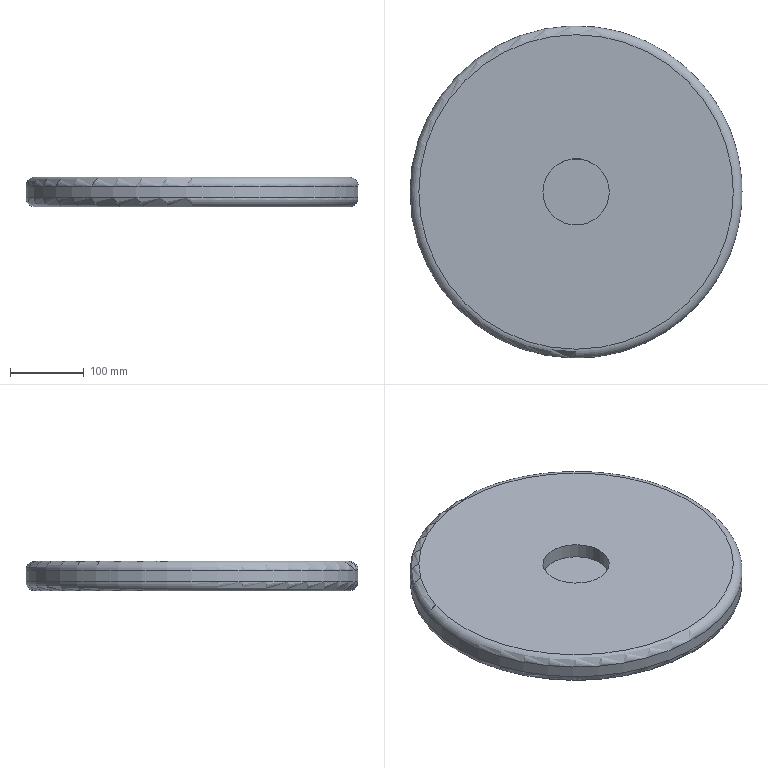Component | NX | BASE | 1 solid | 7 faces | box 450 x 450 x 40 mm | volume 6148156 mm3 | plane 3 | cylinder 2 | torus 2 | commonest cylinder face diameters 450 x1 90 x1
STEP:
#1=CARTESIAN_POINT('',(0.,0.,0.));
#2=DIRECTION('',(0.,0.,1.));
#3=DIRECTION('',(1.,0.,0.));
#4=AXIS2_PLACEMENT_3D('',#1,#2,#3);
#5=CARTESIAN_POINT('',(-225.,-0.,-1130.5));
#6=VERTEX_POINT('',#5);
#7=CARTESIAN_POINT('',(0.,-0.,-1130.5));
#8=DIRECTION('',(0.,0.,1.));
#9=DIRECTION('',(-1.,0.,0.));
#10=AXIS2_PLACEMENT_3D('',#7,#8,#9);
#11=CIRCLE('',#10,225.);
#12=CARTESIAN_POINT('',(0.,-0.,-1102.5));
#13=DIRECTION('',(0.,0.,-1.));
#14=DIRECTION('',(-1.,0.,0.));
#15=AXIS2_PLACEMENT_3D('',#12,#13,#14);
#16=CYLINDRICAL_SURFACE('',#15,225.);
#17=CARTESIAN_POINT('',(6.283,28.));
#18=DIRECTION('',(-1.,0.));
#19=VECTOR('',#18,1.);
#20=LINE('',#17,#19);
#21=(GEOMETRIC_REPRESENTATION_CONTEXT(2)PARAMETRIC_REPRESENTATION_CONTEXT()REPRESENTATION_CONTEXT('',''));
#22=DEFINITIONAL_REPRESENTATION('',(#20),#21);
#23=PCURVE('',#16,#22);
#24=CARTESIAN_POINT('',(0.,-0.,-1130.5));
#25=DIRECTION('',(0.,0.,-1.));
#26=DIRECTION('',(-1.,0.,0.));
#27=AXIS2_PLACEMENT_3D('',#24,#25,#26);
#28=TOROIDAL_SURFACE('',#27,213.,12.);
#29=CARTESIAN_POINT('',(6.283,6.283));
#30=DIRECTION('',(-1.,0.));
#31=VECTOR('',#30,1.);
#32=LINE('',#29,#31);
#33=(GEOMETRIC_REPRESENTATION_CONTEXT(2)PARAMETRIC_REPRESENTATION_CONTEXT()REPRESENTATION_CONTEXT('',''));
#34=DEFINITIONAL_REPRESENTATION('',(#32),#33);
#35=PCURVE('',#28,#34);
#36=SURFACE_CURVE('',#11,(#23,#35),.PCURVE_S1.);
#37=EDGE_CURVE('',#6,#6,#36,.T.);
#38=ORIENTED_EDGE('',*,*,#37,.T.);
#39=CARTESIAN_POINT('',(-225.,-0.,-1114.5));
#40=VERTEX_POINT('',#39);
#41=CARTESIAN_POINT('',(-225.,-0.,-1114.5));
#42=CARTESIAN_POINT('',(-225.,-0.,-1130.5));
#43=B_SPLINE_CURVE_WITH_KNOTS('',1,(#41,#42),.UNSPECIFIED.,.F.,.F.,(2,2),(12.,28.),.PIECEWISE_BEZIER_KNOTS.);
#44=CARTESIAN_POINT('',(0.,0.));
#45=DIRECTION('',(0.,1.));
#46=VECTOR('',#45,1.);
#47=LINE('',#44,#46);
#48=(GEOMETRIC_REPRESENTATION_CONTEXT(2)PARAMETRIC_REPRESENTATION_CONTEXT()REPRESENTATION_CONTEXT('',''));
#49=DEFINITIONAL_REPRESENTATION('',(#47),#48);
#50=PCURVE('',#16,#49);
#51=CARTESIAN_POINT('',(6.283,0.));
#52=DIRECTION('',(0.,1.));
#53=VECTOR('',#52,1.);
#54=LINE('',#51,#53);
#55=(GEOMETRIC_REPRESENTATION_CONTEXT(2)PARAMETRIC_REPRESENTATION_CONTEXT()REPRESENTATION_CONTEXT('',''));
#56=DEFINITIONAL_REPRESENTATION('',(#54),#55);
#57=PCURVE('',#16,#56);
#58=SEAM_CURVE('',#43,(#50,#57),.PCURVE_S1.);
#59=EDGE_CURVE('',#40,#6,#58,.T.);
#60=ORIENTED_EDGE('',*,*,#59,.F.);
#61=CARTESIAN_POINT('',(0.,-0.,-1114.5));
#62=DIRECTION('',(0.,0.,-1.));
#63=DIRECTION('',(-1.,0.,0.));
#64=AXIS2_PLACEMENT_3D('',#61,#62,#63);
#65=CIRCLE('',#64,225.);
#66=CARTESIAN_POINT('',(0.,12.));
#67=DIRECTION('',(1.,0.));
#68=VECTOR('',#67,1.);
#69=LINE('',#66,#68);
#70=(GEOMETRIC_REPRESENTATION_CONTEXT(2)PARAMETRIC_REPRESENTATION_CONTEXT()REPRESENTATION_CONTEXT('',''));
#71=DEFINITIONAL_REPRESENTATION('',(#69),#70);
#72=PCURVE('',#16,#71);
#73=CARTESIAN_POINT('',(0.,-0.,-1114.5));
#74=DIRECTION('',(0.,0.,-1.));
#75=DIRECTION('',(-1.,0.,0.));
#76=AXIS2_PLACEMENT_3D('',#73,#74,#75);
#77=TOROIDAL_SURFACE('',#76,213.,12.);
#78=CARTESIAN_POINT('',(0.,6.283));
#79=DIRECTION('',(1.,0.));
#80=VECTOR('',#79,1.);
#81=LINE('',#78,#80);
#82=(GEOMETRIC_REPRESENTATION_CONTEXT(2)PARAMETRIC_REPRESENTATION_CONTEXT()REPRESENTATION_CONTEXT('',''));
#83=DEFINITIONAL_REPRESENTATION('',(#81),#82);
#84=PCURVE('',#77,#83);
#85=SURFACE_CURVE('',#65,(#72,#84),.PCURVE_S1.);
#86=EDGE_CURVE('',#40,#40,#85,.T.);
#87=ORIENTED_EDGE('',*,*,#86,.T.);
#88=ORIENTED_EDGE('',*,*,#59,.T.);
#89=EDGE_LOOP('',(#38,#60,#87,#88));
#90=FACE_BOUND('',#89,.T.);
#91=ADVANCED_FACE('',(#90),#16,.T.);
#92=CARTESIAN_POINT('',(45.,-0.,-1102.5));
#93=VERTEX_POINT('',#92);
#94=CARTESIAN_POINT('',(0.,-0.,-1102.5));
#95=DIRECTION('',(0.,0.,-1.));
#96=DIRECTION('',(1.,0.,0.));
#97=AXIS2_PLACEMENT_3D('',#94,#95,#96);
#98=CIRCLE('',#97,45.);
#99=CARTESIAN_POINT('',(0.,-0.,-1102.5));
#100=DIRECTION('',(0.,0.,-1.));
#101=DIRECTION('',(-1.,0.,0.));
#102=AXIS2_PLACEMENT_3D('',#99,#100,#101);
#103=PLANE('',#102);
#104=CARTESIAN_POINT('',(0.,0.));
#105=DIRECTION('',(-1.,0.));
#106=AXIS2_PLACEMENT_2D('',#104,#105);
#107=CIRCLE('',#106,45.);
#108=(GEOMETRIC_REPRESENTATION_CONTEXT(2)PARAMETRIC_REPRESENTATION_CONTEXT()REPRESENTATION_CONTEXT('',''));
#109=DEFINITIONAL_REPRESENTATION('',(#107),#108);
#110=PCURVE('',#103,#109);
#111=CARTESIAN_POINT('',(0.,-0.,-1122.5));
#112=DIRECTION('',(0.,0.,1.));
#113=DIRECTION('',(1.,0.,0.));
#114=AXIS2_PLACEMENT_3D('',#111,#112,#113);
#115=CYLINDRICAL_SURFACE('',#114,45.);
#116=CARTESIAN_POINT('',(6.283,20.));
#117=DIRECTION('',(-1.,0.));
#118=VECTOR('',#117,1.);
#119=LINE('',#116,#118);
#120=(GEOMETRIC_REPRESENTATION_CONTEXT(2)PARAMETRIC_REPRESENTATION_CONTEXT()REPRESENTATION_CONTEXT('',''));
#121=DEFINITIONAL_REPRESENTATION('',(#119),#120);
#122=PCURVE('',#115,#121);
#123=SURFACE_CURVE('',#98,(#110,#122),.PCURVE_S1.);
#124=EDGE_CURVE('',#93,#93,#123,.T.);
#125=ORIENTED_EDGE('',*,*,#124,.T.);
#126=EDGE_LOOP('',(#125));
#127=FACE_BOUND('',#126,.T.);
#128=CARTESIAN_POINT('',(-213.,-0.,-1102.5));
#129=VERTEX_POINT('',#128);
#130=CARTESIAN_POINT('',(0.,-0.,-1102.5));
#131=DIRECTION('',(0.,0.,1.));
#132=DIRECTION('',(-1.,0.,0.));
#133=AXIS2_PLACEMENT_3D('',#130,#131,#132);
#134=CIRCLE('',#133,213.);
#135=CARTESIAN_POINT('',(213.,0.));
#136=CARTESIAN_POINT('',(213.,-368.927));
#137=CARTESIAN_POINT('',(-106.5,-184.463));
#138=CARTESIAN_POINT('',(-426.,-0.));
#139=CARTESIAN_POINT('',(-106.5,184.463));
#140=CARTESIAN_POINT('',(213.,368.927));
#141=CARTESIAN_POINT('',(213.,0.));
#142=(BOUNDED_CURVE()B_SPLINE_CURVE(2,(#135,#136,#137,#138,#139,#140,#141),.UNSPECIFIED.,.T.,.F.)B_SPLINE_CURVE_WITH_KNOTS((1,2,2,2,2,1),(-2.094,0.,2.094,4.189,6.283,8.378),.UNSPECIFIED.)CURVE()GEOMETRIC_REPRESENTATION_ITEM()RATIONAL_B_SPLINE_CURVE((1.,0.5,1.,0.5,1.,0.5,1.))REPRESENTATION_ITEM(''));
#143=(GEOMETRIC_REPRESENTATION_CONTEXT(2)PARAMETRIC_REPRESENTATION_CONTEXT()REPRESENTATION_CONTEXT('',''));
#144=DEFINITIONAL_REPRESENTATION('',(#142),#143);
#145=PCURVE('',#103,#144);
#146=CARTESIAN_POINT('',(6.283,4.712));
#147=DIRECTION('',(-1.,0.));
#148=VECTOR('',#147,1.);
#149=LINE('',#146,#148);
#150=(GEOMETRIC_REPRESENTATION_CONTEXT(2)PARAMETRIC_REPRESENTATION_CONTEXT()REPRESENTATION_CONTEXT('',''));
#151=DEFINITIONAL_REPRESENTATION('',(#149),#150);
#152=PCURVE('',#77,#151);
#153=SURFACE_CURVE('',#134,(#145,#152),.PCURVE_S1.);
#154=EDGE_CURVE('',#129,#129,#153,.T.);
#155=ORIENTED_EDGE('',*,*,#154,.T.);
#156=EDGE_LOOP('',(#155));
#157=FACE_BOUND('',#156,.T.);
#158=ADVANCED_FACE('',(#127,#157),#103,.F.);
#159=CARTESIAN_POINT('',(-213.,-0.,-1142.5));
#160=VERTEX_POINT('',#159);
#161=CARTESIAN_POINT('',(0.,-0.,-1142.5));
#162=DIRECTION('',(0.,0.,-1.));
#163=DIRECTION('',(-1.,0.,0.));
#164=AXIS2_PLACEMENT_3D('',#161,#162,#163);
#165=CIRCLE('',#164,213.);
#166=CARTESIAN_POINT('',(0.,-0.,-1142.5));
#167=DIRECTION('',(0.,0.,-1.));
#168=DIRECTION('',(-1.,0.,0.));
#169=AXIS2_PLACEMENT_3D('',#166,#167,#168);
#170=PLANE('',#169);
#171=CARTESIAN_POINT('',(0.,0.));
#172=DIRECTION('',(1.,0.));
#173=AXIS2_PLACEMENT_2D('',#171,#172);
#174=CIRCLE('',#173,213.);
#175=(GEOMETRIC_REPRESENTATION_CONTEXT(2)PARAMETRIC_REPRESENTATION_CONTEXT()REPRESENTATION_CONTEXT('',''));
#176=DEFINITIONAL_REPRESENTATION('',(#174),#175);
#177=PCURVE('',#170,#176);
#178=CARTESIAN_POINT('',(0.,7.854));
#179=DIRECTION('',(1.,0.));
#180=VECTOR('',#179,1.);
#181=LINE('',#178,#180);
#182=(GEOMETRIC_REPRESENTATION_CONTEXT(2)PARAMETRIC_REPRESENTATION_CONTEXT()REPRESENTATION_CONTEXT('',''));
#183=DEFINITIONAL_REPRESENTATION('',(#181),#182);
#184=PCURVE('',#28,#183);
#185=SURFACE_CURVE('',#165,(#177,#184),.PCURVE_S1.);
#186=EDGE_CURVE('',#160,#160,#185,.T.);
#187=ORIENTED_EDGE('',*,*,#186,.T.);
#188=EDGE_LOOP('',(#187));
#189=FACE_BOUND('',#188,.T.);
#190=ADVANCED_FACE('',(#189),#170,.T.);
#191=ORIENTED_EDGE('',*,*,#37,.F.);
#192=CARTESIAN_POINT('',(-225.,-0.,-1130.5));
#193=CARTESIAN_POINT('',(-225.,-0.,-1133.708));
#194=CARTESIAN_POINT('',(-223.98,-0.,-1136.833));
#195=CARTESIAN_POINT('',(-222.023,-0.,-1139.523));
#196=CARTESIAN_POINT('',(-219.333,-0.,-1141.48));
#197=CARTESIAN_POINT('',(-216.208,-0.,-1142.5));
#198=CARTESIAN_POINT('',(-213.,-0.,-1142.5));
#199=(BOUNDED_CURVE()B_SPLINE_CURVE(6,(#192,#193,#194,#195,#196,#197,#198),.UNSPECIFIED.,.F.,.F.)B_SPLINE_CURVE_WITH_KNOTS((7,7),(0.,1.571),.PIECEWISE_BEZIER_KNOTS.)CURVE()GEOMETRIC_REPRESENTATION_ITEM()RATIONAL_B_SPLINE_CURVE((1.031,1.01,0.9979,0.994,0.9979,1.01,1.031))REPRESENTATION_ITEM(''));
#200=CARTESIAN_POINT('',(6.283,6.283));
#201=DIRECTION('',(0.,1.));
#202=VECTOR('',#201,1.);
#203=LINE('',#200,#202);
#204=(GEOMETRIC_REPRESENTATION_CONTEXT(2)PARAMETRIC_REPRESENTATION_CONTEXT()REPRESENTATION_CONTEXT('',''));
#205=DEFINITIONAL_REPRESENTATION('',(#203),#204);
#206=PCURVE('',#28,#205);
#207=CARTESIAN_POINT('',(0.,6.283));
#208=DIRECTION('',(0.,1.));
#209=VECTOR('',#208,1.);
#210=LINE('',#207,#209);
#211=(GEOMETRIC_REPRESENTATION_CONTEXT(2)PARAMETRIC_REPRESENTATION_CONTEXT()REPRESENTATION_CONTEXT('',''));
#212=DEFINITIONAL_REPRESENTATION('',(#210),#211);
#213=PCURVE('',#28,#212);
#214=SEAM_CURVE('',#199,(#206,#213),.PCURVE_S1.);
#215=EDGE_CURVE('',#6,#160,#214,.T.);
#216=ORIENTED_EDGE('',*,*,#215,.T.);
#217=ORIENTED_EDGE('',*,*,#186,.F.);
#218=ORIENTED_EDGE('',*,*,#215,.F.);
#219=EDGE_LOOP('',(#191,#216,#217,#218));
#220=FACE_BOUND('',#219,.T.);
#221=ADVANCED_FACE('',(#220),#28,.T.);
#222=ORIENTED_EDGE('',*,*,#154,.F.);
#223=CARTESIAN_POINT('',(-213.,-0.,-1102.5));
#224=CARTESIAN_POINT('',(-216.208,-0.,-1102.5));
#225=CARTESIAN_POINT('',(-219.333,-0.,-1103.52));
#226=CARTESIAN_POINT('',(-222.023,-0.,-1105.477));
#227=CARTESIAN_POINT('',(-223.98,-0.,-1108.167));
#228=CARTESIAN_POINT('',(-225.,-0.,-1111.292));
#229=CARTESIAN_POINT('',(-225.,-0.,-1114.5));
#230=(BOUNDED_CURVE()B_SPLINE_CURVE(6,(#223,#224,#225,#226,#227,#228,#229),.UNSPECIFIED.,.F.,.F.)B_SPLINE_CURVE_WITH_KNOTS((7,7),(4.712,6.283),.PIECEWISE_BEZIER_KNOTS.)CURVE()GEOMETRIC_REPRESENTATION_ITEM()RATIONAL_B_SPLINE_CURVE((1.031,1.01,0.9979,0.994,0.9979,1.01,1.031))REPRESENTATION_ITEM(''));
#231=CARTESIAN_POINT('',(6.283,0.));
#232=DIRECTION('',(0.,1.));
#233=VECTOR('',#232,1.);
#234=LINE('',#231,#233);
#235=(GEOMETRIC_REPRESENTATION_CONTEXT(2)PARAMETRIC_REPRESENTATION_CONTEXT()REPRESENTATION_CONTEXT('',''));
#236=DEFINITIONAL_REPRESENTATION('',(#234),#235);
#237=PCURVE('',#77,#236);
#238=CARTESIAN_POINT('',(0.,0.));
#239=DIRECTION('',(0.,1.));
#240=VECTOR('',#239,1.);
#241=LINE('',#238,#240);
#242=(GEOMETRIC_REPRESENTATION_CONTEXT(2)PARAMETRIC_REPRESENTATION_CONTEXT()REPRESENTATION_CONTEXT('',''));
#243=DEFINITIONAL_REPRESENTATION('',(#241),#242);
#244=PCURVE('',#77,#243);
#245=SEAM_CURVE('',#230,(#237,#244),.PCURVE_S1.);
#246=EDGE_CURVE('',#129,#40,#245,.T.);
#247=ORIENTED_EDGE('',*,*,#246,.T.);
#248=ORIENTED_EDGE('',*,*,#86,.F.);
#249=ORIENTED_EDGE('',*,*,#246,.F.);
#250=EDGE_LOOP('',(#222,#247,#248,#249));
#251=FACE_BOUND('',#250,.T.);
#252=ADVANCED_FACE('',(#251),#77,.T.);
#253=CARTESIAN_POINT('',(45.,-0.,-1122.5));
#254=VERTEX_POINT('',#253);
#255=CARTESIAN_POINT('',(0.,-0.,-1122.5));
#256=DIRECTION('',(0.,0.,1.));
#257=DIRECTION('',(1.,0.,0.));
#258=AXIS2_PLACEMENT_3D('',#255,#256,#257);
#259=CIRCLE('',#258,45.);
#260=CARTESIAN_POINT('',(0.,0.));
#261=DIRECTION('',(1.,0.));
#262=VECTOR('',#261,1.);
#263=LINE('',#260,#262);
#264=(GEOMETRIC_REPRESENTATION_CONTEXT(2)PARAMETRIC_REPRESENTATION_CONTEXT()REPRESENTATION_CONTEXT('',''));
#265=DEFINITIONAL_REPRESENTATION('',(#263),#264);
#266=PCURVE('',#115,#265);
#267=CARTESIAN_POINT('',(0.,-0.,-1122.5));
#268=DIRECTION('',(0.,0.,-1.));
#269=DIRECTION('',(-1.,0.,0.));
#270=AXIS2_PLACEMENT_3D('',#267,#268,#269);
#271=PLANE('',#270);
#272=CARTESIAN_POINT('',(-45.,0.));
#273=CARTESIAN_POINT('',(-45.,77.942));
#274=CARTESIAN_POINT('',(22.5,38.971));
#275=CARTESIAN_POINT('',(90.,0.));
#276=CARTESIAN_POINT('',(22.5,-38.971));
#277=CARTESIAN_POINT('',(-45.,-77.942));
#278=CARTESIAN_POINT('',(-45.,0.));
#279=(BOUNDED_CURVE()B_SPLINE_CURVE(2,(#272,#273,#274,#275,#276,#277,#278),.UNSPECIFIED.,.T.,.F.)B_SPLINE_CURVE_WITH_KNOTS((1,2,2,2,2,1),(-2.094,0.,2.094,4.189,6.283,8.378),.UNSPECIFIED.)CURVE()GEOMETRIC_REPRESENTATION_ITEM()RATIONAL_B_SPLINE_CURVE((1.,0.5,1.,0.5,1.,0.5,1.))REPRESENTATION_ITEM(''));
#280=(GEOMETRIC_REPRESENTATION_CONTEXT(2)PARAMETRIC_REPRESENTATION_CONTEXT()REPRESENTATION_CONTEXT('',''));
#281=DEFINITIONAL_REPRESENTATION('',(#279),#280);
#282=PCURVE('',#271,#281);
#283=SURFACE_CURVE('',#259,(#266,#282),.PCURVE_S1.);
#284=EDGE_CURVE('',#254,#254,#283,.T.);
#285=ORIENTED_EDGE('',*,*,#284,.T.);
#286=CARTESIAN_POINT('',(45.,-0.,-1122.5));
#287=CARTESIAN_POINT('',(45.,-0.,-1102.5));
#288=B_SPLINE_CURVE_WITH_KNOTS('',1,(#286,#287),.UNSPECIFIED.,.F.,.F.,(2,2),(0.,20.),.PIECEWISE_BEZIER_KNOTS.);
#289=CARTESIAN_POINT('',(6.283,0.));
#290=DIRECTION('',(0.,1.));
#291=VECTOR('',#290,1.);
#292=LINE('',#289,#291);
#293=(GEOMETRIC_REPRESENTATION_CONTEXT(2)PARAMETRIC_REPRESENTATION_CONTEXT()REPRESENTATION_CONTEXT('',''));
#294=DEFINITIONAL_REPRESENTATION('',(#292),#293);
#295=PCURVE('',#115,#294);
#296=CARTESIAN_POINT('',(0.,0.));
#297=DIRECTION('',(0.,1.));
#298=VECTOR('',#297,1.);
#299=LINE('',#296,#298);
#300=(GEOMETRIC_REPRESENTATION_CONTEXT(2)PARAMETRIC_REPRESENTATION_CONTEXT()REPRESENTATION_CONTEXT('',''));
#301=DEFINITIONAL_REPRESENTATION('',(#299),#300);
#302=PCURVE('',#115,#301);
#303=SEAM_CURVE('',#288,(#295,#302),.PCURVE_S1.);
#304=EDGE_CURVE('',#254,#93,#303,.T.);
#305=ORIENTED_EDGE('',*,*,#304,.T.);
#306=ORIENTED_EDGE('',*,*,#124,.T.);
#307=ORIENTED_EDGE('',*,*,#304,.F.);
#308=EDGE_LOOP('',(#285,#305,#306,#307));
#309=FACE_BOUND('',#308,.F.);
#310=ADVANCED_FACE('',(#309),#115,.F.);
#311=ORIENTED_EDGE('',*,*,#284,.T.);
#312=EDGE_LOOP('',(#311));
#313=FACE_BOUND('',#312,.T.);
#314=ADVANCED_FACE('',(#313),#271,.F.);
#315=CLOSED_SHELL('',(#91,#158,#190,#221,#252,#310,#314));
#316=MANIFOLD_SOLID_BREP('',#315);
#317=(LENGTH_UNIT()NAMED_UNIT(*)SI_UNIT(.MILLI.,.METRE.));
#318=UNCERTAINTY_MEASURE_WITH_UNIT(LENGTH_MEASURE(0.00001),#317,'','');
#319=(NAMED_UNIT(*)PLANE_ANGLE_UNIT()SI_UNIT($,.RADIAN.));
#320=(NAMED_UNIT(*)SI_UNIT($,.STERADIAN.)SOLID_ANGLE_UNIT());
#321=(GEOMETRIC_REPRESENTATION_CONTEXT(3)GLOBAL_UNCERTAINTY_ASSIGNED_CONTEXT((#318))GLOBAL_UNIT_ASSIGNED_CONTEXT((#317,#319,#320))REPRESENTATION_CONTEXT('',''));
#322=ADVANCED_BREP_SHAPE_REPRESENTATION('',(#4,#316),#321);